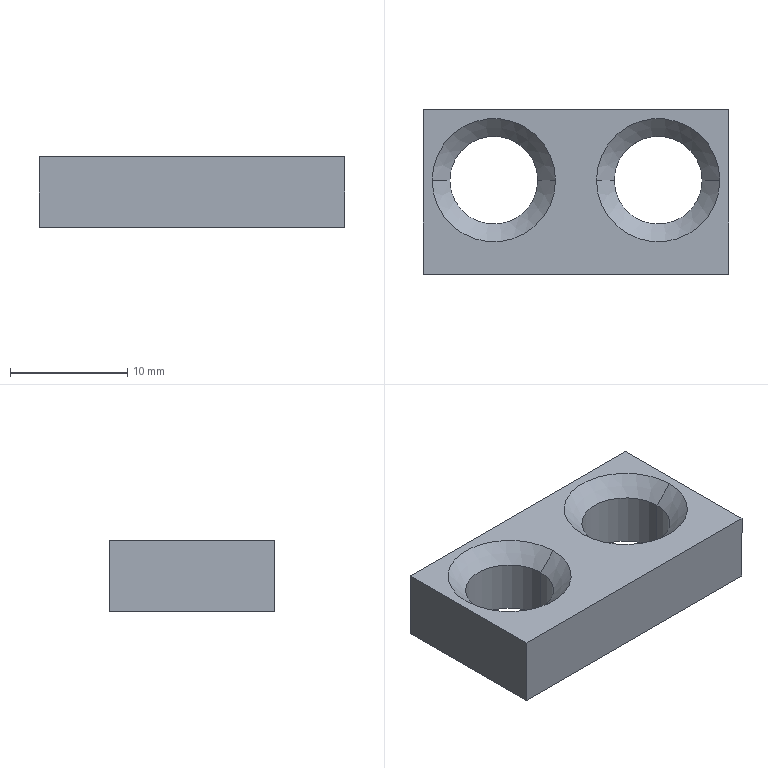Component | SolidWorks | 30PressureBlock-1 | 1 solid | 14 faces | box 26 x 14 x 6 mm | volume 1594 mm3 | plane 6 | cone 4 | cylinder 4 | commonest cylinder face diameters 7.5 x4
build123d program:
from build123d import *

# Parameters (mm, degrees)
SKETCH1_W           = 26
SKETCH1_H           = 14
BOSS_EXTRUDE1_DEPTH = 6
HOLE1_AT_2_COUNT    = 2
HOLE1_AT_2_PITCH    = 14
CHAMFER1_SIZE       = 1.5


with BuildPart() as part:
    # Sketch1 → Boss-Extrude1 (new body)
    with BuildSketch(Plane.XY):
        Rectangle(SKETCH1_W, SKETCH1_H)
    extrude(amount=BOSS_EXTRUDE1_DEPTH)

    # Sketch3 → Hole1 (revolve, cut)
    with BuildSketch(Plane(origin=(-7, -1, 6), x_dir=(0, -1, 0), z_dir=(1, 0, 0))):
        Polygon((0, 0), (0, 14), (3.75, 14), (3.75, -1.5), (2.25, 0), align=None)
    hole1 = revolve(axis=Axis((-7, -1, 12.445), (0, 0, -1)), mode=Mode.SUBTRACT)

    # Hole1 at 2: Hole1 ×2
    with Locations(*[(i * HOLE1_AT_2_PITCH, 0, 0) for i in range(1, HOLE1_AT_2_COUNT)]):
        add(hole1, mode=Mode.SUBTRACT)

    # Chamfer1
    chamfer1_edges = [part.edges().sort_by_distance(p)[0] for p in [
        (-7, 2.75, 6),
        (7, 2.75, 6),
    ]]
    chamfer(chamfer1_edges, length=CHAMFER1_SIZE)


solid = part.part

# Placed as in the assembly
solid = solid.moved(Location((10.191, 33, -92), (0, 0, 180)))
STEP:
#1=COLOUR_RGB('',0.7922,0.8196,0.9333);
#2=FILL_AREA_STYLE_COLOUR('',#1);
#3=FILL_AREA_STYLE('',(#2));
#4=SURFACE_STYLE_FILL_AREA(#3);
#5=SURFACE_SIDE_STYLE('',(#4));
#6=SURFACE_STYLE_USAGE(.BOTH.,#5);
#7=PRESENTATION_STYLE_ASSIGNMENT((#6));
#8=CARTESIAN_POINT('',(0.8244,1.339,-3.445));
#9=VERTEX_POINT('',#8);
#10=CARTESIAN_POINT('',(0.5292,1.339,-3.445));
#11=VERTEX_POINT('',#10);
#12=CARTESIAN_POINT('',(0.6768,1.339,-3.445));
#13=DIRECTION('',(0.,0.,1.));
#14=DIRECTION('',(-1.,0.,0.));
#15=AXIS2_PLACEMENT_3D('',#12,#13,#14);
#16=CIRCLE('',#15,0.1476);
#17=EDGE_CURVE('',#9,#11,#16,.T.);
#18=ORIENTED_EDGE('',*,*,#17,.F.);
#19=CARTESIAN_POINT('',(0.8835,1.339,-3.386));
#20=VERTEX_POINT('',#19);
#21=CARTESIAN_POINT('',(0.8244,1.339,-3.445));
#22=DIRECTION('',(0.7071,0.,0.7071));
#23=VECTOR('',#22,39.37);
#24=LINE('',#21,#23);
#25=EDGE_CURVE('',#9,#20,#24,.T.);
#26=ORIENTED_EDGE('',*,*,#25,.T.);
#27=CARTESIAN_POINT('',(0.4701,1.339,-3.386));
#28=VERTEX_POINT('',#27);
#29=CARTESIAN_POINT('',(0.6768,1.339,-3.386));
#30=DIRECTION('',(-0.,-0.,-1.));
#31=DIRECTION('',(-1.,0.,0.));
#32=AXIS2_PLACEMENT_3D('',#29,#30,#31);
#33=CIRCLE('',#32,0.2067);
#34=EDGE_CURVE('',#28,#20,#33,.T.);
#35=ORIENTED_EDGE('',*,*,#34,.F.);
#36=CARTESIAN_POINT('',(0.5292,1.339,-3.445));
#37=DIRECTION('',(-0.7071,0.,0.7071));
#38=VECTOR('',#37,39.37);
#39=LINE('',#36,#38);
#40=EDGE_CURVE('',#11,#28,#39,.T.);
#41=ORIENTED_EDGE('',*,*,#40,.F.);
#42=EDGE_LOOP('',(#18,#26,#35,#41));
#43=FACE_OUTER_BOUND('',#42,.T.);
#44=CARTESIAN_POINT('',(0.6768,1.339,-3.445));
#45=DIRECTION('',(0.,0.,1.));
#46=DIRECTION('',(-1.,0.,0.));
#47=AXIS2_PLACEMENT_3D('',#44,#45,#46);
#48=CONICAL_SURFACE('',#47,0.1476,0.7854);
#49=ADVANCED_FACE('',(#43),#48,.F.);
#50=CARTESIAN_POINT('',(0.2733,1.339,-3.445));
#51=VERTEX_POINT('',#50);
#52=CARTESIAN_POINT('',(-0.02201,1.339,-3.445));
#53=VERTEX_POINT('',#52);
#54=CARTESIAN_POINT('',(0.1256,1.339,-3.445));
#55=DIRECTION('',(0.,0.,1.));
#56=DIRECTION('',(-1.,0.,0.));
#57=AXIS2_PLACEMENT_3D('',#54,#55,#56);
#58=CIRCLE('',#57,0.1476);
#59=EDGE_CURVE('',#51,#53,#58,.T.);
#60=ORIENTED_EDGE('',*,*,#59,.F.);
#61=CARTESIAN_POINT('',(0.3323,1.339,-3.386));
#62=VERTEX_POINT('',#61);
#63=CARTESIAN_POINT('',(0.2733,1.339,-3.445));
#64=DIRECTION('',(0.7071,0.,0.7071));
#65=VECTOR('',#64,39.37);
#66=LINE('',#63,#65);
#67=EDGE_CURVE('',#51,#62,#66,.T.);
#68=ORIENTED_EDGE('',*,*,#67,.T.);
#69=CARTESIAN_POINT('',(-0.08107,1.339,-3.386));
#70=VERTEX_POINT('',#69);
#71=CARTESIAN_POINT('',(0.1256,1.339,-3.386));
#72=DIRECTION('',(-0.,-0.,-1.));
#73=DIRECTION('',(-1.,0.,0.));
#74=AXIS2_PLACEMENT_3D('',#71,#72,#73);
#75=CIRCLE('',#74,0.2067);
#76=EDGE_CURVE('',#70,#62,#75,.T.);
#77=ORIENTED_EDGE('',*,*,#76,.F.);
#78=CARTESIAN_POINT('',(-0.02201,1.339,-3.445));
#79=DIRECTION('',(-0.7071,0.,0.7071));
#80=VECTOR('',#79,39.37);
#81=LINE('',#78,#80);
#82=EDGE_CURVE('',#53,#70,#81,.T.);
#83=ORIENTED_EDGE('',*,*,#82,.F.);
#84=EDGE_LOOP('',(#60,#68,#77,#83));
#85=FACE_OUTER_BOUND('',#84,.T.);
#86=CARTESIAN_POINT('',(0.1256,1.339,-3.445));
#87=DIRECTION('',(0.,0.,1.));
#88=DIRECTION('',(-1.,0.,0.));
#89=AXIS2_PLACEMENT_3D('',#86,#87,#88);
#90=CONICAL_SURFACE('',#89,0.1476,0.7854);
#91=ADVANCED_FACE('',(#85),#90,.F.);
#92=CARTESIAN_POINT('',(0.2733,1.339,-3.622));
#93=VERTEX_POINT('',#92);
#94=CARTESIAN_POINT('',(-0.02201,1.339,-3.622));
#95=VERTEX_POINT('',#94);
#96=CARTESIAN_POINT('',(0.1256,1.339,-3.622));
#97=DIRECTION('',(0.,0.,1.));
#98=DIRECTION('',(-1.,0.,0.));
#99=AXIS2_PLACEMENT_3D('',#96,#97,#98);
#100=CIRCLE('',#99,0.1476);
#101=EDGE_CURVE('',#93,#95,#100,.T.);
#102=ORIENTED_EDGE('',*,*,#101,.F.);
#103=CARTESIAN_POINT('',(0.2733,1.339,-3.386));
#104=DIRECTION('',(0.,0.,1.));
#105=VECTOR('',#104,39.37);
#106=LINE('',#103,#105);
#107=EDGE_CURVE('',#93,#51,#106,.T.);
#108=ORIENTED_EDGE('',*,*,#107,.T.);
#109=ORIENTED_EDGE('',*,*,#59,.T.);
#110=CARTESIAN_POINT('',(-0.02201,1.339,-3.386));
#111=DIRECTION('',(0.,0.,1.));
#112=VECTOR('',#111,39.37);
#113=LINE('',#110,#112);
#114=EDGE_CURVE('',#95,#53,#113,.T.);
#115=ORIENTED_EDGE('',*,*,#114,.F.);
#116=EDGE_LOOP('',(#102,#108,#109,#115));
#117=FACE_OUTER_BOUND('',#116,.T.);
#118=CARTESIAN_POINT('',(0.1256,1.339,-3.386));
#119=DIRECTION('',(0.,0.,1.));
#120=DIRECTION('',(-1.,0.,0.));
#121=AXIS2_PLACEMENT_3D('',#118,#119,#120);
#122=CYLINDRICAL_SURFACE('',#121,0.1476);
#123=ADVANCED_FACE('',(#117),#122,.F.);
#124=CARTESIAN_POINT('',(0.8244,1.339,-3.622));
#125=VERTEX_POINT('',#124);
#126=CARTESIAN_POINT('',(0.5292,1.339,-3.622));
#127=VERTEX_POINT('',#126);
#128=CARTESIAN_POINT('',(0.6768,1.339,-3.622));
#129=DIRECTION('',(0.,0.,1.));
#130=DIRECTION('',(-1.,0.,0.));
#131=AXIS2_PLACEMENT_3D('',#128,#129,#130);
#132=CIRCLE('',#131,0.1476);
#133=EDGE_CURVE('',#125,#127,#132,.T.);
#134=ORIENTED_EDGE('',*,*,#133,.F.);
#135=CARTESIAN_POINT('',(0.8244,1.339,-3.386));
#136=DIRECTION('',(0.,0.,1.));
#137=VECTOR('',#136,39.37);
#138=LINE('',#135,#137);
#139=EDGE_CURVE('',#125,#9,#138,.T.);
#140=ORIENTED_EDGE('',*,*,#139,.T.);
#141=ORIENTED_EDGE('',*,*,#17,.T.);
#142=CARTESIAN_POINT('',(0.5292,1.339,-3.386));
#143=DIRECTION('',(0.,0.,1.));
#144=VECTOR('',#143,39.37);
#145=LINE('',#142,#144);
#146=EDGE_CURVE('',#127,#11,#145,.T.);
#147=ORIENTED_EDGE('',*,*,#146,.F.);
#148=EDGE_LOOP('',(#134,#140,#141,#147));
#149=FACE_OUTER_BOUND('',#148,.T.);
#150=CARTESIAN_POINT('',(0.6768,1.339,-3.386));
#151=DIRECTION('',(0.,0.,1.));
#152=DIRECTION('',(-1.,0.,0.));
#153=AXIS2_PLACEMENT_3D('',#150,#151,#152);
#154=CYLINDRICAL_SURFACE('',#153,0.1476);
#155=ADVANCED_FACE('',(#149),#154,.F.);
#156=ORIENTED_EDGE('',*,*,#76,.T.);
#157=CARTESIAN_POINT('',(0.1256,1.339,-3.386));
#158=DIRECTION('',(-0.,-0.,-1.));
#159=DIRECTION('',(-1.,0.,0.));
#160=AXIS2_PLACEMENT_3D('',#157,#158,#159);
#161=CIRCLE('',#160,0.2067);
#162=EDGE_CURVE('',#62,#70,#161,.T.);
#163=ORIENTED_EDGE('',*,*,#162,.T.);
#164=EDGE_LOOP('',(#156,#163));
#165=FACE_BOUND('',#164,.T.);
#166=ORIENTED_EDGE('',*,*,#34,.T.);
#167=CARTESIAN_POINT('',(0.6768,1.339,-3.386));
#168=DIRECTION('',(-0.,-0.,-1.));
#169=DIRECTION('',(-1.,0.,0.));
#170=AXIS2_PLACEMENT_3D('',#167,#168,#169);
#171=CIRCLE('',#170,0.2067);
#172=EDGE_CURVE('',#20,#28,#171,.T.);
#173=ORIENTED_EDGE('',*,*,#172,.T.);
#174=EDGE_LOOP('',(#166,#173));
#175=FACE_BOUND('',#174,.T.);
#176=CARTESIAN_POINT('',(-0.1106,1.575,-3.386));
#177=VERTEX_POINT('',#176);
#178=CARTESIAN_POINT('',(-0.1106,1.024,-3.386));
#179=VERTEX_POINT('',#178);
#180=CARTESIAN_POINT('',(-0.1106,1.024,-3.386));
#181=DIRECTION('',(0.,-1.,0.));
#182=VECTOR('',#181,39.37);
#183=LINE('',#180,#182);
#184=EDGE_CURVE('',#177,#179,#183,.T.);
#185=ORIENTED_EDGE('',*,*,#184,.T.);
#186=CARTESIAN_POINT('',(0.913,1.024,-3.386));
#187=VERTEX_POINT('',#186);
#188=CARTESIAN_POINT('',(0.913,1.024,-3.386));
#189=DIRECTION('',(1.,-0.,-0.));
#190=VECTOR('',#189,39.37);
#191=LINE('',#188,#190);
#192=EDGE_CURVE('',#179,#187,#191,.T.);
#193=ORIENTED_EDGE('',*,*,#192,.T.);
#194=CARTESIAN_POINT('',(0.913,1.575,-3.386));
#195=VERTEX_POINT('',#194);
#196=CARTESIAN_POINT('',(0.913,1.024,-3.386));
#197=DIRECTION('',(-0.,1.,-0.));
#198=VECTOR('',#197,39.37);
#199=LINE('',#196,#198);
#200=EDGE_CURVE('',#187,#195,#199,.T.);
#201=ORIENTED_EDGE('',*,*,#200,.T.);
#202=CARTESIAN_POINT('',(0.913,1.575,-3.386));
#203=DIRECTION('',(-1.,0.,0.));
#204=VECTOR('',#203,39.37);
#205=LINE('',#202,#204);
#206=EDGE_CURVE('',#195,#177,#205,.T.);
#207=ORIENTED_EDGE('',*,*,#206,.T.);
#208=EDGE_LOOP('',(#185,#193,#201,#207));
#209=FACE_OUTER_BOUND('',#208,.T.);
#210=CARTESIAN_POINT('',(0.4012,1.299,-3.386));
#211=DIRECTION('',(0.,0.,1.));
#212=DIRECTION('',(-1.,0.,0.));
#213=AXIS2_PLACEMENT_3D('',#210,#211,#212);
#214=PLANE('',#213);
#215=ADVANCED_FACE('',(#165,#175,#209),#214,.T.);
#216=CARTESIAN_POINT('',(-0.1106,1.575,-3.622));
#217=VERTEX_POINT('',#216);
#218=CARTESIAN_POINT('',(-0.1106,1.024,-3.622));
#219=VERTEX_POINT('',#218);
#220=CARTESIAN_POINT('',(-0.1106,1.024,-3.622));
#221=DIRECTION('',(0.,-1.,0.));
#222=VECTOR('',#221,39.37);
#223=LINE('',#220,#222);
#224=EDGE_CURVE('',#217,#219,#223,.T.);
#225=ORIENTED_EDGE('',*,*,#224,.T.);
#226=CARTESIAN_POINT('',(-0.1106,1.024,-3.386));
#227=DIRECTION('',(-0.,-0.,-1.));
#228=VECTOR('',#227,39.37);
#229=LINE('',#226,#228);
#230=EDGE_CURVE('',#179,#219,#229,.T.);
#231=ORIENTED_EDGE('',*,*,#230,.F.);
#232=ORIENTED_EDGE('',*,*,#184,.F.);
#233=CARTESIAN_POINT('',(-0.1106,1.575,-3.386));
#234=DIRECTION('',(-0.,-0.,-1.));
#235=VECTOR('',#234,39.37);
#236=LINE('',#233,#235);
#237=EDGE_CURVE('',#177,#217,#236,.T.);
#238=ORIENTED_EDGE('',*,*,#237,.T.);
#239=EDGE_LOOP('',(#225,#231,#232,#238));
#240=FACE_OUTER_BOUND('',#239,.T.);
#241=CARTESIAN_POINT('',(-0.1106,1.024,-3.386));
#242=DIRECTION('',(1.,0.,-0.));
#243=DIRECTION('',(-0.,1.,-0.));
#244=AXIS2_PLACEMENT_3D('',#241,#242,#243);
#245=PLANE('',#244);
#246=ADVANCED_FACE('',(#240),#245,.F.);
#247=CARTESIAN_POINT('',(0.913,1.024,-3.622));
#248=VERTEX_POINT('',#247);
#249=CARTESIAN_POINT('',(0.913,1.024,-3.622));
#250=DIRECTION('',(1.,-0.,-0.));
#251=VECTOR('',#250,39.37);
#252=LINE('',#249,#251);
#253=EDGE_CURVE('',#219,#248,#252,.T.);
#254=ORIENTED_EDGE('',*,*,#253,.T.);
#255=CARTESIAN_POINT('',(0.913,1.024,-3.386));
#256=DIRECTION('',(-0.,-0.,-1.));
#257=VECTOR('',#256,39.37);
#258=LINE('',#255,#257);
#259=EDGE_CURVE('',#187,#248,#258,.T.);
#260=ORIENTED_EDGE('',*,*,#259,.F.);
#261=ORIENTED_EDGE('',*,*,#192,.F.);
#262=ORIENTED_EDGE('',*,*,#230,.T.);
#263=EDGE_LOOP('',(#254,#260,#261,#262));
#264=FACE_OUTER_BOUND('',#263,.T.);
#265=CARTESIAN_POINT('',(0.913,1.024,-3.386));
#266=DIRECTION('',(0.,1.,-0.));
#267=DIRECTION('',(-0.,-0.,-1.));
#268=AXIS2_PLACEMENT_3D('',#265,#266,#267);
#269=PLANE('',#268);
#270=ADVANCED_FACE('',(#264),#269,.F.);
#271=CARTESIAN_POINT('',(0.913,1.575,-3.622));
#272=VERTEX_POINT('',#271);
#273=CARTESIAN_POINT('',(0.913,1.024,-3.622));
#274=DIRECTION('',(-0.,1.,-0.));
#275=VECTOR('',#274,39.37);
#276=LINE('',#273,#275);
#277=EDGE_CURVE('',#248,#272,#276,.T.);
#278=ORIENTED_EDGE('',*,*,#277,.T.);
#279=CARTESIAN_POINT('',(0.913,1.575,-3.386));
#280=DIRECTION('',(-0.,-0.,-1.));
#281=VECTOR('',#280,39.37);
#282=LINE('',#279,#281);
#283=EDGE_CURVE('',#195,#272,#282,.T.);
#284=ORIENTED_EDGE('',*,*,#283,.F.);
#285=ORIENTED_EDGE('',*,*,#200,.F.);
#286=ORIENTED_EDGE('',*,*,#259,.T.);
#287=EDGE_LOOP('',(#278,#284,#285,#286));
#288=FACE_OUTER_BOUND('',#287,.T.);
#289=CARTESIAN_POINT('',(0.913,1.024,-3.386));
#290=DIRECTION('',(-1.,-0.,0.));
#291=DIRECTION('',(0.,-1.,0.));
#292=AXIS2_PLACEMENT_3D('',#289,#290,#291);
#293=PLANE('',#292);
#294=ADVANCED_FACE('',(#288),#293,.F.);
#295=CARTESIAN_POINT('',(0.913,1.575,-3.622));
#296=DIRECTION('',(-1.,0.,0.));
#297=VECTOR('',#296,39.37);
#298=LINE('',#295,#297);
#299=EDGE_CURVE('',#272,#217,#298,.T.);
#300=ORIENTED_EDGE('',*,*,#299,.T.);
#301=ORIENTED_EDGE('',*,*,#237,.F.);
#302=ORIENTED_EDGE('',*,*,#206,.F.);
#303=ORIENTED_EDGE('',*,*,#283,.T.);
#304=EDGE_LOOP('',(#300,#301,#302,#303));
#305=FACE_OUTER_BOUND('',#304,.T.);
#306=CARTESIAN_POINT('',(0.913,1.575,-3.386));
#307=DIRECTION('',(-0.,-1.,0.));
#308=DIRECTION('',(0.,0.,1.));
#309=AXIS2_PLACEMENT_3D('',#306,#307,#308);
#310=PLANE('',#309);
#311=ADVANCED_FACE('',(#305),#310,.F.);
#312=CARTESIAN_POINT('',(0.1256,1.339,-3.622));
#313=DIRECTION('',(0.,0.,1.));
#314=DIRECTION('',(-1.,0.,0.));
#315=AXIS2_PLACEMENT_3D('',#312,#313,#314);
#316=CIRCLE('',#315,0.1476);
#317=EDGE_CURVE('',#95,#93,#316,.T.);
#318=ORIENTED_EDGE('',*,*,#317,.T.);
#319=ORIENTED_EDGE('',*,*,#101,.T.);
#320=EDGE_LOOP('',(#318,#319));
#321=FACE_BOUND('',#320,.T.);
#322=CARTESIAN_POINT('',(0.6768,1.339,-3.622));
#323=DIRECTION('',(0.,0.,1.));
#324=DIRECTION('',(-1.,0.,0.));
#325=AXIS2_PLACEMENT_3D('',#322,#323,#324);
#326=CIRCLE('',#325,0.1476);
#327=EDGE_CURVE('',#127,#125,#326,.T.);
#328=ORIENTED_EDGE('',*,*,#327,.T.);
#329=ORIENTED_EDGE('',*,*,#133,.T.);
#330=EDGE_LOOP('',(#328,#329));
#331=FACE_BOUND('',#330,.T.);
#332=ORIENTED_EDGE('',*,*,#224,.F.);
#333=ORIENTED_EDGE('',*,*,#299,.F.);
#334=ORIENTED_EDGE('',*,*,#277,.F.);
#335=ORIENTED_EDGE('',*,*,#253,.F.);
#336=EDGE_LOOP('',(#332,#333,#334,#335));
#337=FACE_OUTER_BOUND('',#336,.T.);
#338=CARTESIAN_POINT('',(0.4012,1.299,-3.622));
#339=DIRECTION('',(0.,0.,1.));
#340=DIRECTION('',(-1.,0.,0.));
#341=AXIS2_PLACEMENT_3D('',#338,#339,#340);
#342=PLANE('',#341);
#343=ADVANCED_FACE('',(#321,#331,#337),#342,.F.);
#344=ORIENTED_EDGE('',*,*,#139,.F.);
#345=ORIENTED_EDGE('',*,*,#327,.F.);
#346=ORIENTED_EDGE('',*,*,#146,.T.);
#347=CARTESIAN_POINT('',(0.6768,1.339,-3.445));
#348=DIRECTION('',(0.,0.,1.));
#349=DIRECTION('',(-1.,0.,0.));
#350=AXIS2_PLACEMENT_3D('',#347,#348,#349);
#351=CIRCLE('',#350,0.1476);
#352=EDGE_CURVE('',#11,#9,#351,.T.);
#353=ORIENTED_EDGE('',*,*,#352,.T.);
#354=EDGE_LOOP('',(#344,#345,#346,#353));
#355=FACE_OUTER_BOUND('',#354,.T.);
#356=CARTESIAN_POINT('',(0.6768,1.339,-3.386));
#357=DIRECTION('',(0.,0.,1.));
#358=DIRECTION('',(-1.,0.,0.));
#359=AXIS2_PLACEMENT_3D('',#356,#357,#358);
#360=CYLINDRICAL_SURFACE('',#359,0.1476);
#361=ADVANCED_FACE('',(#355),#360,.F.);
#362=ORIENTED_EDGE('',*,*,#107,.F.);
#363=ORIENTED_EDGE('',*,*,#317,.F.);
#364=ORIENTED_EDGE('',*,*,#114,.T.);
#365=CARTESIAN_POINT('',(0.1256,1.339,-3.445));
#366=DIRECTION('',(0.,0.,1.));
#367=DIRECTION('',(-1.,0.,0.));
#368=AXIS2_PLACEMENT_3D('',#365,#366,#367);
#369=CIRCLE('',#368,0.1476);
#370=EDGE_CURVE('',#53,#51,#369,.T.);
#371=ORIENTED_EDGE('',*,*,#370,.T.);
#372=EDGE_LOOP('',(#362,#363,#364,#371));
#373=FACE_OUTER_BOUND('',#372,.T.);
#374=CARTESIAN_POINT('',(0.1256,1.339,-3.386));
#375=DIRECTION('',(0.,0.,1.));
#376=DIRECTION('',(-1.,0.,0.));
#377=AXIS2_PLACEMENT_3D('',#374,#375,#376);
#378=CYLINDRICAL_SURFACE('',#377,0.1476);
#379=ADVANCED_FACE('',(#373),#378,.F.);
#380=ORIENTED_EDGE('',*,*,#67,.F.);
#381=ORIENTED_EDGE('',*,*,#370,.F.);
#382=ORIENTED_EDGE('',*,*,#82,.T.);
#383=ORIENTED_EDGE('',*,*,#162,.F.);
#384=EDGE_LOOP('',(#380,#381,#382,#383));
#385=FACE_OUTER_BOUND('',#384,.T.);
#386=CARTESIAN_POINT('',(0.1256,1.339,-3.445));
#387=DIRECTION('',(0.,0.,1.));
#388=DIRECTION('',(-1.,0.,0.));
#389=AXIS2_PLACEMENT_3D('',#386,#387,#388);
#390=CONICAL_SURFACE('',#389,0.1476,0.7854);
#391=ADVANCED_FACE('',(#385),#390,.F.);
#392=ORIENTED_EDGE('',*,*,#25,.F.);
#393=ORIENTED_EDGE('',*,*,#352,.F.);
#394=ORIENTED_EDGE('',*,*,#40,.T.);
#395=ORIENTED_EDGE('',*,*,#172,.F.);
#396=EDGE_LOOP('',(#392,#393,#394,#395));
#397=FACE_OUTER_BOUND('',#396,.T.);
#398=CARTESIAN_POINT('',(0.6768,1.339,-3.445));
#399=DIRECTION('',(0.,0.,1.));
#400=DIRECTION('',(-1.,0.,0.));
#401=AXIS2_PLACEMENT_3D('',#398,#399,#400);
#402=CONICAL_SURFACE('',#401,0.1476,0.7854);
#403=ADVANCED_FACE('',(#397),#402,.F.);
#404=CLOSED_SHELL('',(#49,#91,#123,#155,#215,#246,#270,#294,#311,#343,#361,#379,#391,#403));
#405=MANIFOLD_SOLID_BREP('',#404);
#406=STYLED_ITEM('',(#7),#405);
#407=PRESENTATION_LAYER_ASSIGNMENT('','',(#406));
#408=CARTESIAN_POINT('',(0.,0.,0.));
#409=DIRECTION('',(0.,0.,1.));
#410=DIRECTION('',(1.,0.,0.));
#411=AXIS2_PLACEMENT_3D('',#408,#409,#410);
#412=(LENGTH_UNIT()NAMED_UNIT(*)SI_UNIT($,.METRE.));
#413=LENGTH_MEASURE_WITH_UNIT(LENGTH_MEASURE(0.0254),#412);
#414=DIMENSIONAL_EXPONENTS(1.,0.,0.,0.,0.,0.,0.);
#415=(CONVERSION_BASED_UNIT('',#413)LENGTH_UNIT()NAMED_UNIT(#414));
#416=UNCERTAINTY_MEASURE_WITH_UNIT(LENGTH_MEASURE(0.00001),#415,'','');
#417=(NAMED_UNIT(*)PLANE_ANGLE_UNIT()SI_UNIT($,.RADIAN.));
#418=(NAMED_UNIT(*)SI_UNIT($,.STERADIAN.)SOLID_ANGLE_UNIT());
#419=(GEOMETRIC_REPRESENTATION_CONTEXT(3)GLOBAL_UNCERTAINTY_ASSIGNED_CONTEXT((#416))GLOBAL_UNIT_ASSIGNED_CONTEXT((#415,#417,#418))REPRESENTATION_CONTEXT('',''));
#420=ADVANCED_BREP_SHAPE_REPRESENTATION('',(#405,#411),#419);
#421=(LENGTH_UNIT()NAMED_UNIT(*)SI_UNIT($,.METRE.));
#422=LENGTH_MEASURE_WITH_UNIT(LENGTH_MEASURE(0.0254),#421);
#423=DIMENSIONAL_EXPONENTS(1.,0.,0.,0.,0.,0.,0.);
#424=(CONVERSION_BASED_UNIT('',#422)LENGTH_UNIT()NAMED_UNIT(#423));
#425=UNCERTAINTY_MEASURE_WITH_UNIT(LENGTH_MEASURE(0.00001),#424,'','');
#426=(NAMED_UNIT(*)PLANE_ANGLE_UNIT()SI_UNIT($,.RADIAN.));
#427=(NAMED_UNIT(*)SI_UNIT($,.STERADIAN.)SOLID_ANGLE_UNIT());
#428=(GEOMETRIC_REPRESENTATION_CONTEXT(3)GLOBAL_UNCERTAINTY_ASSIGNED_CONTEXT((#425))GLOBAL_UNIT_ASSIGNED_CONTEXT((#424,#426,#427))REPRESENTATION_CONTEXT('',''));
#429=MECHANICAL_DESIGN_GEOMETRIC_PRESENTATION_REPRESENTATION('',(#406),#428);